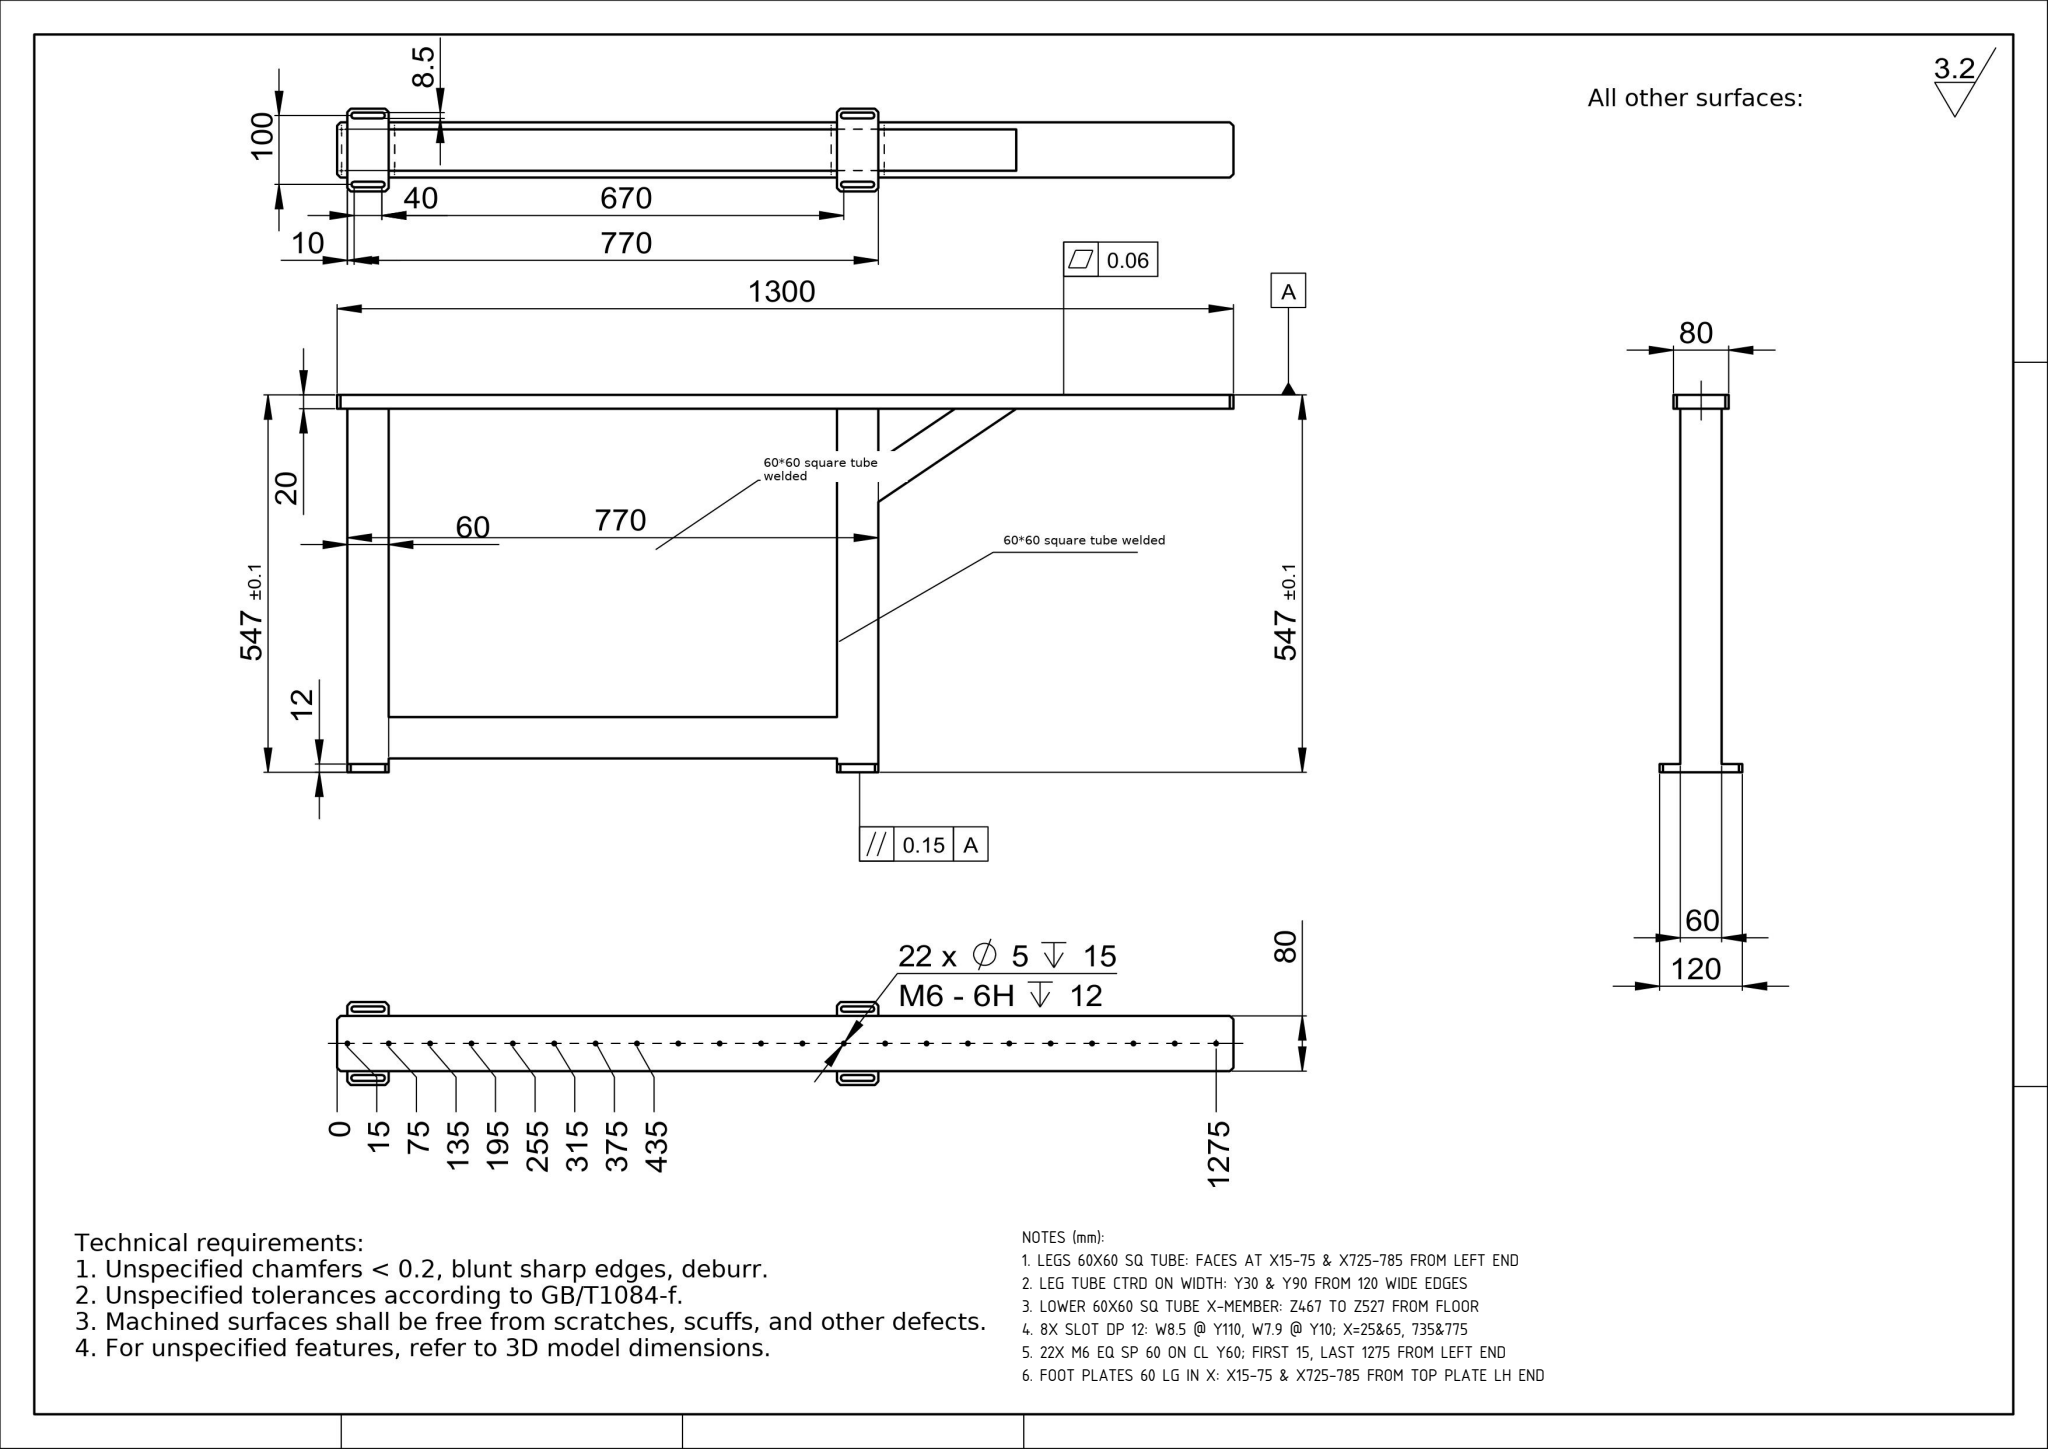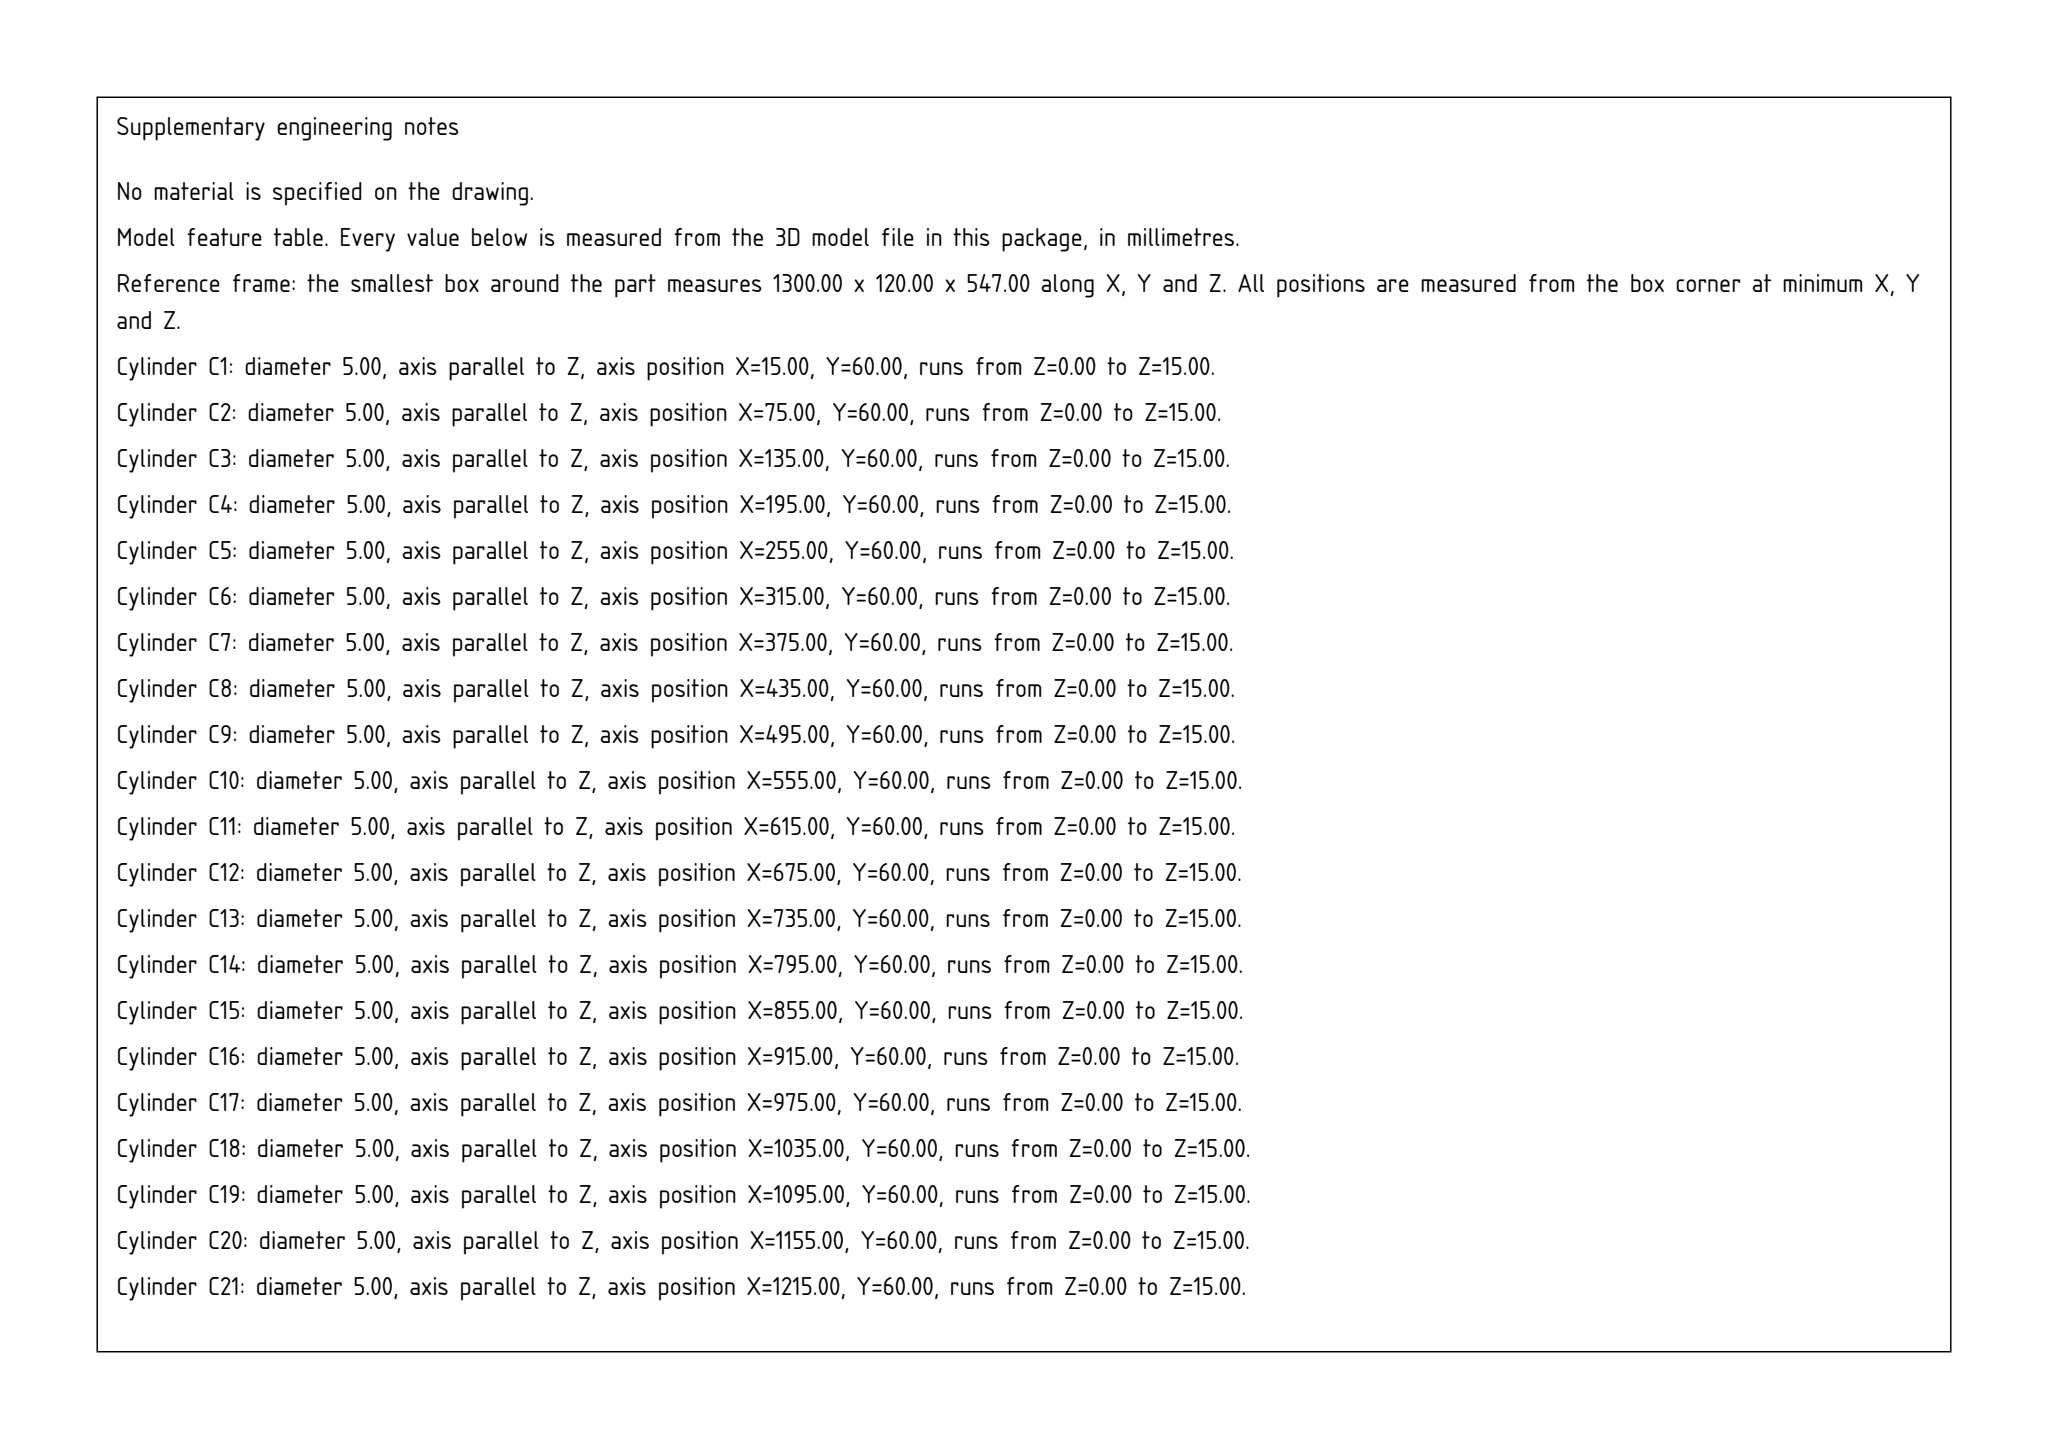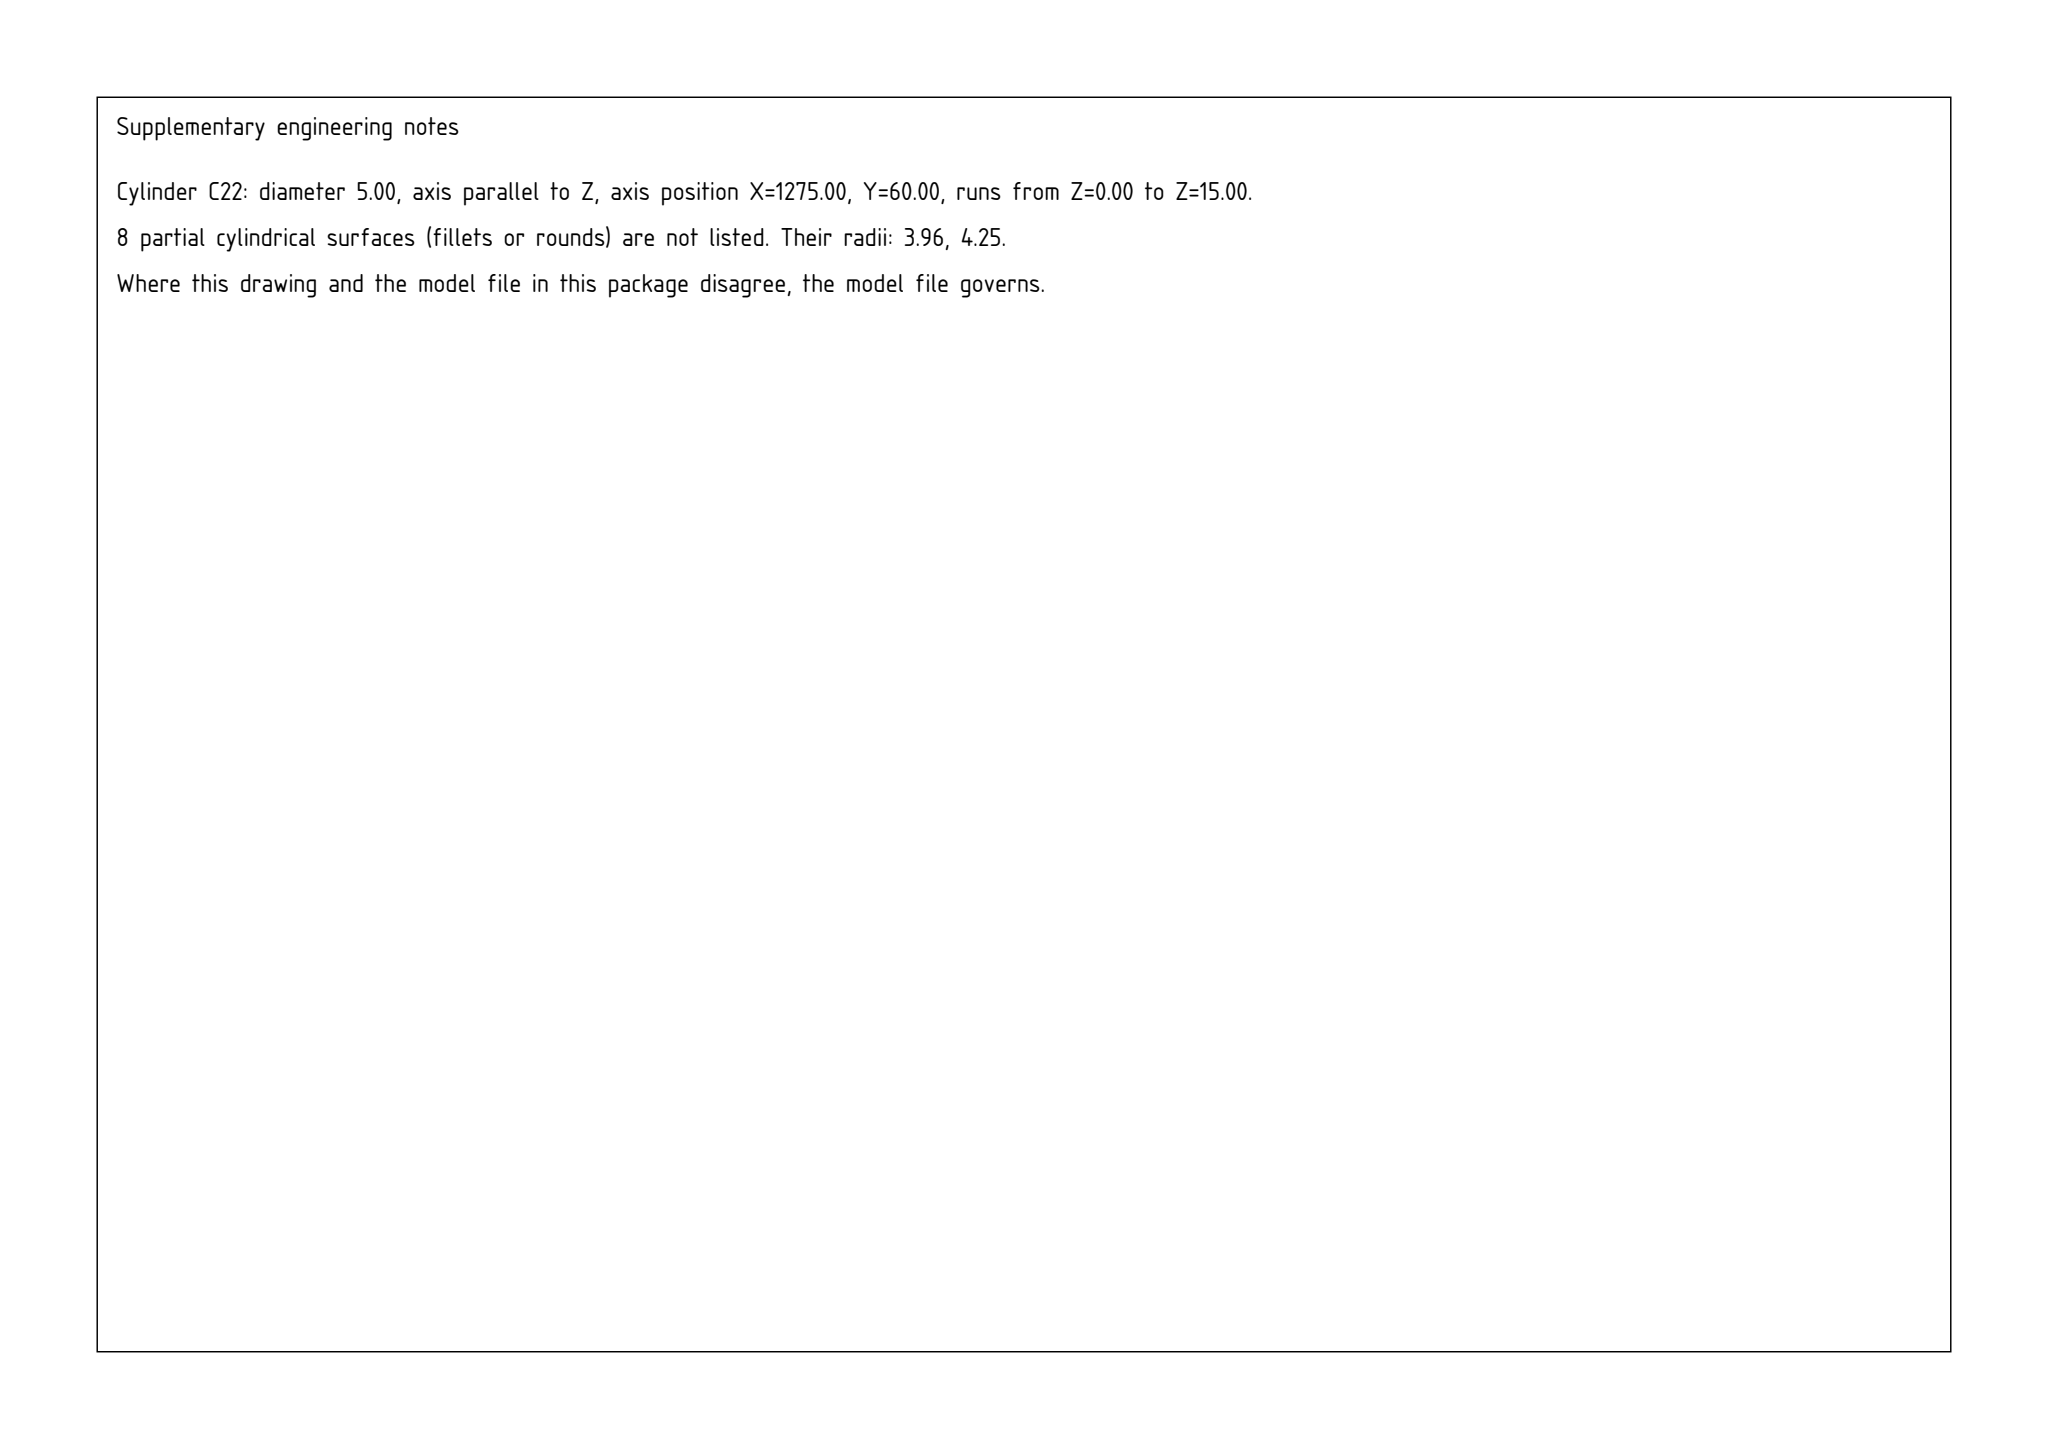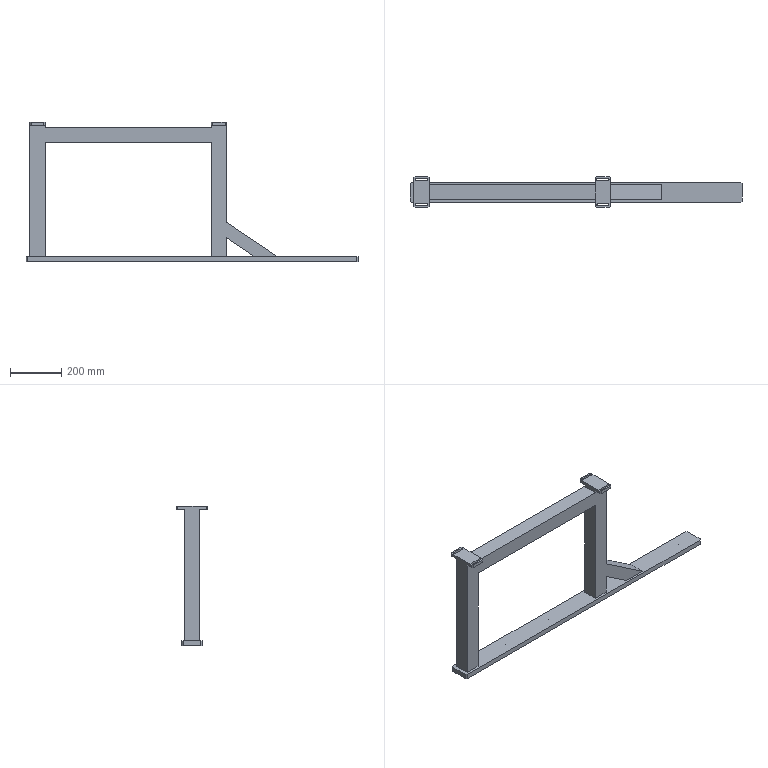Part | SolidWorks | mm | 1 solid | 149 faces | box 1300 x 120 x 547 mm | volume 8833604 mm3 | cylinder 56 | plane 49 | cone 44 | commonest cylinder face diameters 5 x44 8.5 x6 7.914 x6
Drawing notes:
LEGS 60X60 SQ TUBE: FACES AT X15-75 & X725-785 FROM LEFT END | from the solid: x-planes 15,75,725,785; bbox x=1300
LEG TUBE CTRD ON WIDTH: Y30 & Y90 FROM 120 WIDE EDGES | from the solid: y-planes 30 and 90 bounding leg tube in 120 wide bbox
LOWER 60X60 SQ TUBE X-MEMBER: Z467 TO Z527 FROM FLOOR | from the solid: z-planes 467 and 527 (60 apart) between leg faces x=75 & x=725
8X SLOT DP 12: W8.5 @ Y110, W7.9 @ Y10; X=25&65, 735&775 | from the solid: z-holes Ø8.5 at y110 and Ø7.914 at y10, x=25,65,735,775, L=12; y-planes 6.04/13.96 & 105.75/114.25
22X M6 EQ SP 60 ON CL Y60; FIRST 15, LAST 1275 FROM LEFT END | from the solid: Ø5 z-holes at x=15,75,...,1275 (22 pcs), all at y=60.0 of 120 wide bbox
FOOT PLATES 60 LG IN X: X15-75 & X725-785 FROM TOP PLATE LH END | from the solid: x-planes 15/75 and 725/785 bound foot plates (y 0-120, z 0-20); hole slots at x25/65 & x735/775 give 10 and 40 dims; 785-15=770
build123d program:
from build123d import *

# Parameters (mm, degrees)
SKETCH1_W           = 1300
SKETCH1_H           = 80
BOSS_EXTRUDE1_DEPTH = 20
SKETCH2_W           = 60
SKETCH2_H           = 60
BOSS_EXTRUDE2_DEPTH = 515
SKETCH3_W           = 60
SKETCH3_H           = 120
BOSS_EXTRUDE3_DEPTH = 12
CHAMFER1_SIZE       = 5
LPATTERN2_COUNT     = 22
LPATTERN2_PITCH     = 60
SKETCH9_W           = 650
SKETCH9_H           = 60
BOSS_EXTRUDE4_DEPTH = 60
LPATTERN3_COUNT     = 2
LPATTERN3_PITCH     = 710
CHAMFER2_SIZE       = 5
CUT_EXTRUDE1_DEPTH  = 60
LPATTERN4_COUNT     = 2
LPATTERN4_PITCH     = 710
BOSS_EXTRUDE5_DEPTH = 60


with BuildPart() as part:
    # Sketch1 → Boss-Extrude1 (new body)
    with BuildSketch(Plane.XY):
        Rectangle(SKETCH1_W, SKETCH1_H)
    extrude(amount=BOSS_EXTRUDE1_DEPTH)

    # Sketch2 → Boss-Extrude2 (add)
    with BuildSketch(Plane.XY.offset(20)):
        with Locations((-605, 0)):
            Rectangle(SKETCH2_W, SKETCH2_H)
        with Locations((105, 0)):
            Rectangle(SKETCH2_W, SKETCH2_H)
    extrude(amount=BOSS_EXTRUDE2_DEPTH)

    # Sketch3 → Boss-Extrude3 (add)
    with BuildSketch(Plane.XY.offset(535)):
        with Locations((-605, 0)):
            Rectangle(SKETCH3_W, SKETCH3_H)
    boss_extrude3 = extrude(amount=BOSS_EXTRUDE3_DEPTH)

    # Chamfer1
    chamfer1_edges = [part.edges().sort_by_distance(p)[0] for p in [
        (650, -40, 10),
        (-650, -40, 10),
        (-650, 40, 10),
        (650, 40, 10),
    ]]
    chamfer(chamfer1_edges, length=CHAMFER1_SIZE)

    # Sketch8 → M6 Tapped Hole1 (revolve, cut)
    with BuildSketch(Plane.YZ.offset(-635)):
        Polygon((0, 0), (0, 16.502), (2.5, 15), (2.5, 0), align=None)
    m6_tapped_hole1 = revolve(axis=Axis((-635, 0, -6.35), (0, 0, 1)), mode=Mode.SUBTRACT)

    # LPattern2: M6 Tapped Hole1 ×22
    with Locations(*[(i * LPATTERN2_PITCH, 0, 0) for i in range(1, LPATTERN2_COUNT)]):
        add(m6_tapped_hole1, mode=Mode.SUBTRACT)

    # Sketch9 → Boss-Extrude4 (add)
    with BuildSketch(Plane(origin=(0, 30, 0), x_dir=(1, 0, 0), z_dir=(0, 1, 0))):
        with Locations((-250, -497)):
            Rectangle(SKETCH9_W, SKETCH9_H)
    extrude(amount=-BOSS_EXTRUDE4_DEPTH)

    # LPattern3: Boss-Extrude3 ×2
    with Locations(*[(i * LPATTERN3_PITCH, 0, 0) for i in range(1, LPATTERN3_COUNT)]):
        add(boss_extrude3)

    # Chamfer2
    chamfer2_edges = [part.edges().sort_by_distance(p)[0] for p in [
        (75, 60, 541),
        (75, -60, 541),
        (135, -60, 541),
        (135, 60, 541),
        (-635, 60, 541),
        (-635, -60, 541),
        (-575, -60, 541),
        (-575, 60, 541),
    ]]
    chamfer(chamfer2_edges, length=CHAMFER2_SIZE)

    # Sketch10 → Cut-Extrude1 (cut)
    with BuildSketch(Plane.XY.offset(547)):
        with BuildLine():
            Line((85, 54.25), (125, 54.25))
            ThreePointArc((125, 54.25), (129.25, 50), (125, 45.75))
            Line((125, 45.75), (85, 45.75))
            ThreePointArc((85, 45.75), (80.75, 50), (85, 54.25))
        make_face()
        with BuildLine():
            Line((85, -46.043), (125, -46.043))
            ThreePointArc((125, -46.043), (128.957, -50), (125, -53.957))
            Line((125, -53.957), (85, -53.957))
            ThreePointArc((85, -53.957), (81.043, -50), (85, -46.043))
        make_face()
    cut_extrude1 = extrude(amount=-CUT_EXTRUDE1_DEPTH, mode=Mode.SUBTRACT)

    # LPattern4: Cut-Extrude1 ×2
    with Locations(*[(-i * LPATTERN4_PITCH, 0, 0) for i in range(1, LPATTERN4_COUNT)]):
        add(cut_extrude1, mode=Mode.SUBTRACT)

    # Sketch11 → Boss-Extrude5 (add)
    with BuildSketch(Plane(origin=(0, 30, 0), x_dir=(1, 0, 0), z_dir=(0, 1, 0))):
        Polygon((135, -95), (246.111, -20), (335, -20), (135, -155), align=None)
    extrude(amount=-BOSS_EXTRUDE5_DEPTH)


solid = part.part